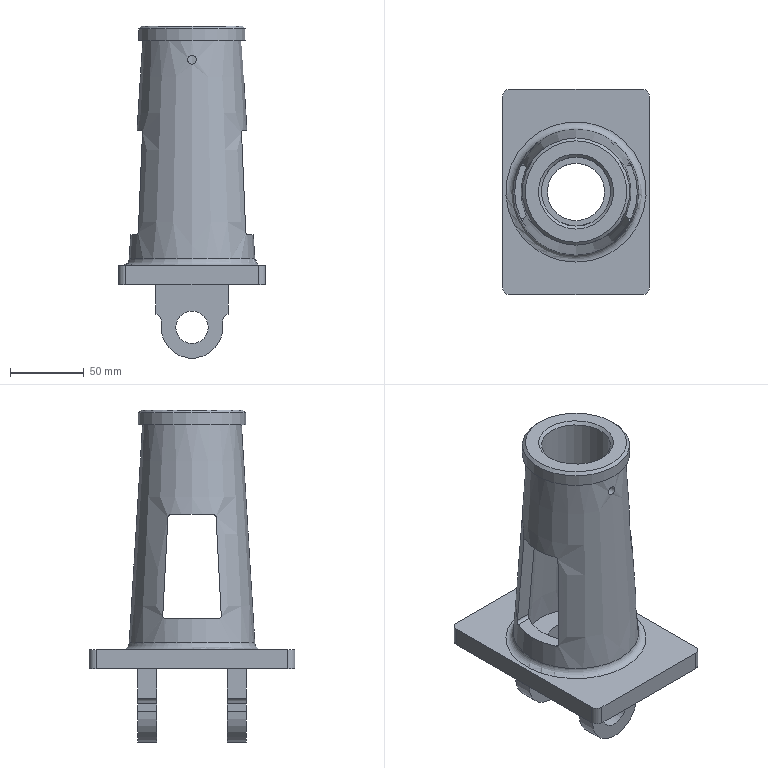Component | NX | MACHINEBODY | 1 solid | 59 faces | volume 497670 mm3 | plane 30 | cylinder 24 | cone 4 | torus 1 | commonest cylinder face diameters 4 x8 10 x4 8 x4 42 x2 22 x2 47 x1 73 x1 39 x1